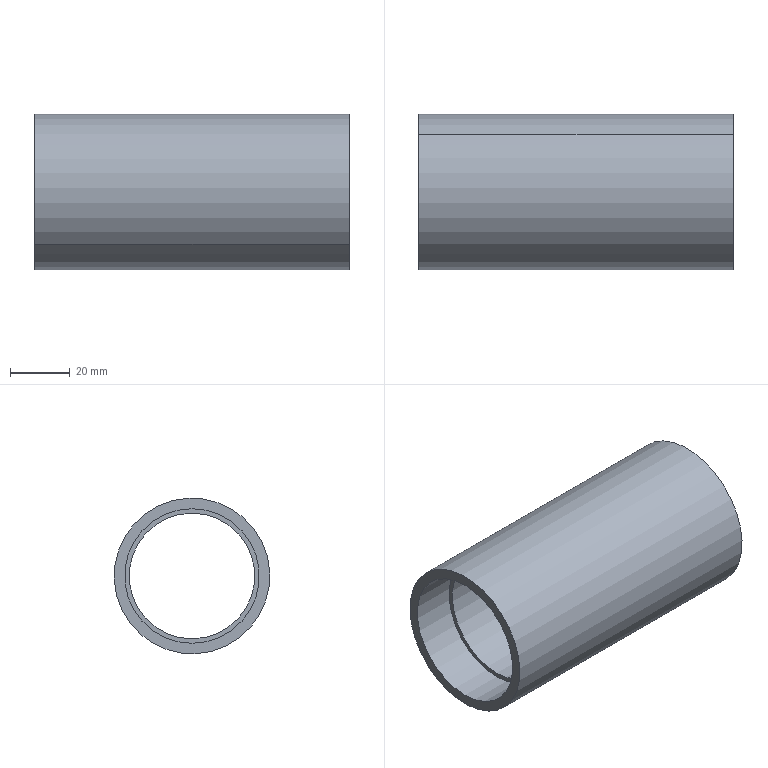Component | SolidWorks | GuideMechanism-1_EncoderRoller-1 | 1 solid | 12 faces | box 105 x 52 x 52 mm | volume 71369 mm3 | cylinder 8 | plane 4 | commonest cylinder face diameters 45 x4 52 x2 42 x2
build123d program:
from build123d import *

# Parameters (mm, degrees)
SKETCH1_W          = 20
SKETCH1_H          = 105
SKETCH2_R          = 21
CUT_EXTRUDE1_DEPTH = 112.252
SKETCH3_R          = 22.5
CUT_EXTRUDE2_DEPTH = 15
CUT_EXTRUDE3_START = -15
SKETCH4_R          = 22.5
CUT_EXTRUDE3_DEPTH = 15


with BuildPart() as part:
    # Sketch1 → Revolve1 (revolve)
    with BuildSketch(Plane.XY):
        with Locations((16, 52.5)):
            Rectangle(SKETCH1_W, SKETCH1_H)
    revolve(axis=Axis((0, -318.491, 0), (0, 1, 0)))

    # Sketch2 → Cut-Extrude1 (cut, through all)
    with BuildSketch(Plane.XZ):
        Circle(SKETCH2_R)
    extrude(amount=-CUT_EXTRUDE1_DEPTH, mode=Mode.SUBTRACT)

    # Sketch3 → Cut-Extrude2 (cut)
    with BuildSketch(Plane.XZ):
        Circle(SKETCH3_R)
    extrude(amount=-CUT_EXTRUDE2_DEPTH, mode=Mode.SUBTRACT)

    # Sketch4 → Cut-Extrude3 (cut)
    with BuildSketch(Plane(origin=(0, 105, 0), x_dir=(1, 0, 0), z_dir=(0, 1, 0)).offset(CUT_EXTRUDE3_START)):
        Circle(SKETCH4_R)
    extrude(amount=CUT_EXTRUDE3_DEPTH, mode=Mode.SUBTRACT)


solid = part.part

# Placed as in the assembly
solid = solid.moved(Location((-386.772, -352.564, 1209.912), (0, 0, 90)))
STEP:
#1=COLOUR_RGB('',0.7922,0.8196,0.9333);
#2=FILL_AREA_STYLE_COLOUR('',#1);
#3=FILL_AREA_STYLE('',(#2));
#4=SURFACE_STYLE_FILL_AREA(#3);
#5=SURFACE_SIDE_STYLE('',(#4));
#6=SURFACE_STYLE_USAGE(.BOTH.,#5);
#7=PRESENTATION_STYLE_ASSIGNMENT((#6));
#8=CARTESIAN_POINT('',(-15.818,-14.538,47.041));
#9=VERTEX_POINT('',#8);
#10=CARTESIAN_POINT('',(-15.818,-13.223,48.227));
#11=VERTEX_POINT('',#10);
#12=CARTESIAN_POINT('',(-15.818,-13.88,47.634));
#13=DIRECTION('',(1.,0.,0.));
#14=DIRECTION('',(0.,0.7428,0.6696));
#15=AXIS2_PLACEMENT_3D('',#12,#13,#14);
#16=CIRCLE('',#15,0.8858);
#17=EDGE_CURVE('',#9,#11,#16,.T.);
#18=ORIENTED_EDGE('',*,*,#17,.F.);
#19=CARTESIAN_POINT('',(-15.227,-14.538,47.041));
#20=VERTEX_POINT('',#19);
#21=CARTESIAN_POINT('',(-15.818,-14.538,47.041));
#22=DIRECTION('',(1.,0.,0.));
#23=VECTOR('',#22,39.37);
#24=LINE('',#21,#23);
#25=EDGE_CURVE('',#9,#20,#24,.T.);
#26=ORIENTED_EDGE('',*,*,#25,.T.);
#27=CARTESIAN_POINT('',(-15.227,-13.223,48.227));
#28=VERTEX_POINT('',#27);
#29=CARTESIAN_POINT('',(-15.227,-13.88,47.634));
#30=DIRECTION('',(1.,0.,0.));
#31=DIRECTION('',(0.,0.7428,0.6696));
#32=AXIS2_PLACEMENT_3D('',#29,#30,#31);
#33=CIRCLE('',#32,0.8858);
#34=EDGE_CURVE('',#20,#28,#33,.T.);
#35=ORIENTED_EDGE('',*,*,#34,.T.);
#36=CARTESIAN_POINT('',(-15.818,-13.223,48.227));
#37=DIRECTION('',(1.,0.,0.));
#38=VECTOR('',#37,39.37);
#39=LINE('',#36,#38);
#40=EDGE_CURVE('',#11,#28,#39,.T.);
#41=ORIENTED_EDGE('',*,*,#40,.F.);
#42=EDGE_LOOP('',(#18,#26,#35,#41));
#43=FACE_OUTER_BOUND('',#42,.T.);
#44=CARTESIAN_POINT('',(-15.818,-13.88,47.634));
#45=DIRECTION('',(1.,0.,0.));
#46=DIRECTION('',(0.,0.7428,0.6696));
#47=AXIS2_PLACEMENT_3D('',#44,#45,#46);
#48=CYLINDRICAL_SURFACE('',#47,0.8858);
#49=ADVANCED_FACE('',(#43),#48,.F.);
#50=CARTESIAN_POINT('',(-18.771,-13.223,48.227));
#51=VERTEX_POINT('',#50);
#52=CARTESIAN_POINT('',(-18.771,-14.538,47.041));
#53=VERTEX_POINT('',#52);
#54=CARTESIAN_POINT('',(-18.771,-13.88,47.634));
#55=DIRECTION('',(-1.,-0.,-0.));
#56=DIRECTION('',(0.,-0.7428,-0.6696));
#57=AXIS2_PLACEMENT_3D('',#54,#55,#56);
#58=CIRCLE('',#57,0.8858);
#59=EDGE_CURVE('',#51,#53,#58,.T.);
#60=ORIENTED_EDGE('',*,*,#59,.F.);
#61=CARTESIAN_POINT('',(-19.361,-13.223,48.227));
#62=VERTEX_POINT('',#61);
#63=CARTESIAN_POINT('',(-18.771,-13.223,48.227));
#64=DIRECTION('',(-1.,-0.,-0.));
#65=VECTOR('',#64,39.37);
#66=LINE('',#63,#65);
#67=EDGE_CURVE('',#51,#62,#66,.T.);
#68=ORIENTED_EDGE('',*,*,#67,.T.);
#69=CARTESIAN_POINT('',(-19.361,-14.538,47.041));
#70=VERTEX_POINT('',#69);
#71=CARTESIAN_POINT('',(-19.361,-13.88,47.634));
#72=DIRECTION('',(-1.,-0.,-0.));
#73=DIRECTION('',(0.,-0.7428,-0.6696));
#74=AXIS2_PLACEMENT_3D('',#71,#72,#73);
#75=CIRCLE('',#74,0.8858);
#76=EDGE_CURVE('',#62,#70,#75,.T.);
#77=ORIENTED_EDGE('',*,*,#76,.T.);
#78=CARTESIAN_POINT('',(-18.771,-14.538,47.041));
#79=DIRECTION('',(-1.,-0.,-0.));
#80=VECTOR('',#79,39.37);
#81=LINE('',#78,#80);
#82=EDGE_CURVE('',#53,#70,#81,.T.);
#83=ORIENTED_EDGE('',*,*,#82,.F.);
#84=EDGE_LOOP('',(#60,#68,#77,#83));
#85=FACE_OUTER_BOUND('',#84,.T.);
#86=CARTESIAN_POINT('',(-18.771,-13.88,47.634));
#87=DIRECTION('',(-1.,-0.,-0.));
#88=DIRECTION('',(0.,-0.7428,-0.6696));
#89=AXIS2_PLACEMENT_3D('',#86,#87,#88);
#90=CYLINDRICAL_SURFACE('',#89,0.8858);
#91=ADVANCED_FACE('',(#85),#90,.F.);
#92=CARTESIAN_POINT('',(-15.227,-14.641,46.949));
#93=VERTEX_POINT('',#92);
#94=CARTESIAN_POINT('',(-15.227,-13.12,48.32));
#95=VERTEX_POINT('',#94);
#96=CARTESIAN_POINT('',(-15.227,-13.88,47.634));
#97=DIRECTION('',(-1.,-0.,-0.));
#98=DIRECTION('',(0.,-0.7428,-0.6696));
#99=AXIS2_PLACEMENT_3D('',#96,#97,#98);
#100=CIRCLE('',#99,1.024);
#101=EDGE_CURVE('',#93,#95,#100,.T.);
#102=ORIENTED_EDGE('',*,*,#101,.T.);
#103=CARTESIAN_POINT('',(-19.361,-13.12,48.32));
#104=VERTEX_POINT('',#103);
#105=CARTESIAN_POINT('',(-31.9,-13.12,48.32));
#106=DIRECTION('',(-1.,-0.,-0.));
#107=VECTOR('',#106,39.37);
#108=LINE('',#105,#107);
#109=EDGE_CURVE('',#95,#104,#108,.T.);
#110=ORIENTED_EDGE('',*,*,#109,.T.);
#111=CARTESIAN_POINT('',(-19.361,-14.641,46.949));
#112=VERTEX_POINT('',#111);
#113=CARTESIAN_POINT('',(-19.361,-13.88,47.634));
#114=DIRECTION('',(-1.,-0.,-0.));
#115=DIRECTION('',(0.,-0.7428,-0.6696));
#116=AXIS2_PLACEMENT_3D('',#113,#114,#115);
#117=CIRCLE('',#116,1.024);
#118=EDGE_CURVE('',#112,#104,#117,.T.);
#119=ORIENTED_EDGE('',*,*,#118,.F.);
#120=CARTESIAN_POINT('',(-31.9,-14.641,46.949));
#121=DIRECTION('',(-1.,-0.,-0.));
#122=VECTOR('',#121,39.37);
#123=LINE('',#120,#122);
#124=EDGE_CURVE('',#93,#112,#123,.T.);
#125=ORIENTED_EDGE('',*,*,#124,.F.);
#126=EDGE_LOOP('',(#102,#110,#119,#125));
#127=FACE_OUTER_BOUND('',#126,.T.);
#128=CARTESIAN_POINT('',(-31.9,-13.88,47.634));
#129=DIRECTION('',(-1.,-0.,-0.));
#130=DIRECTION('',(0.,-0.7428,-0.6696));
#131=AXIS2_PLACEMENT_3D('',#128,#129,#130);
#132=CYLINDRICAL_SURFACE('',#131,1.024);
#133=ADVANCED_FACE('',(#127),#132,.T.);
#134=CARTESIAN_POINT('',(-15.818,-13.266,48.188));
#135=VERTEX_POINT('',#134);
#136=CARTESIAN_POINT('',(-15.818,-14.495,47.081));
#137=VERTEX_POINT('',#136);
#138=CARTESIAN_POINT('',(-15.818,-13.88,47.634));
#139=DIRECTION('',(-1.,-0.,-0.));
#140=DIRECTION('',(0.,0.7428,0.6696));
#141=AXIS2_PLACEMENT_3D('',#138,#139,#140);
#142=CIRCLE('',#141,0.8268);
#143=EDGE_CURVE('',#135,#137,#142,.T.);
#144=ORIENTED_EDGE('',*,*,#143,.F.);
#145=CARTESIAN_POINT('',(-18.771,-13.266,48.188));
#146=VERTEX_POINT('',#145);
#147=CARTESIAN_POINT('',(-15.227,-13.266,48.188));
#148=DIRECTION('',(-1.,-0.,-0.));
#149=VECTOR('',#148,39.37);
#150=LINE('',#147,#149);
#151=EDGE_CURVE('',#135,#146,#150,.T.);
#152=ORIENTED_EDGE('',*,*,#151,.T.);
#153=CARTESIAN_POINT('',(-18.771,-14.495,47.081));
#154=VERTEX_POINT('',#153);
#155=CARTESIAN_POINT('',(-18.771,-13.88,47.634));
#156=DIRECTION('',(1.,0.,0.));
#157=DIRECTION('',(0.,-0.7428,-0.6696));
#158=AXIS2_PLACEMENT_3D('',#155,#156,#157);
#159=CIRCLE('',#158,0.8268);
#160=EDGE_CURVE('',#154,#146,#159,.T.);
#161=ORIENTED_EDGE('',*,*,#160,.F.);
#162=CARTESIAN_POINT('',(-15.227,-14.495,47.081));
#163=DIRECTION('',(-1.,-0.,-0.));
#164=VECTOR('',#163,39.37);
#165=LINE('',#162,#164);
#166=EDGE_CURVE('',#137,#154,#165,.T.);
#167=ORIENTED_EDGE('',*,*,#166,.F.);
#168=EDGE_LOOP('',(#144,#152,#161,#167));
#169=FACE_OUTER_BOUND('',#168,.T.);
#170=CARTESIAN_POINT('',(-15.227,-13.88,47.634));
#171=DIRECTION('',(-1.,-0.,-0.));
#172=DIRECTION('',(0.,-0.7428,-0.6696));
#173=AXIS2_PLACEMENT_3D('',#170,#171,#172);
#174=CYLINDRICAL_SURFACE('',#173,0.8268);
#175=ADVANCED_FACE('',(#169),#174,.F.);
#176=ORIENTED_EDGE('',*,*,#151,.F.);
#177=CARTESIAN_POINT('',(-15.818,-13.88,47.634));
#178=DIRECTION('',(-1.,-0.,-0.));
#179=DIRECTION('',(0.,0.7428,0.6696));
#180=AXIS2_PLACEMENT_3D('',#177,#178,#179);
#181=CIRCLE('',#180,0.8268);
#182=EDGE_CURVE('',#137,#135,#181,.T.);
#183=ORIENTED_EDGE('',*,*,#182,.F.);
#184=ORIENTED_EDGE('',*,*,#166,.T.);
#185=CARTESIAN_POINT('',(-18.771,-13.88,47.634));
#186=DIRECTION('',(1.,0.,0.));
#187=DIRECTION('',(0.,-0.7428,-0.6696));
#188=AXIS2_PLACEMENT_3D('',#185,#186,#187);
#189=CIRCLE('',#188,0.8268);
#190=EDGE_CURVE('',#146,#154,#189,.T.);
#191=ORIENTED_EDGE('',*,*,#190,.F.);
#192=EDGE_LOOP('',(#176,#183,#184,#191));
#193=FACE_OUTER_BOUND('',#192,.T.);
#194=CARTESIAN_POINT('',(-15.227,-13.88,47.634));
#195=DIRECTION('',(-1.,-0.,-0.));
#196=DIRECTION('',(0.,-0.7428,-0.6696));
#197=AXIS2_PLACEMENT_3D('',#194,#195,#196);
#198=CYLINDRICAL_SURFACE('',#197,0.8268);
#199=ADVANCED_FACE('',(#193),#198,.F.);
#200=CARTESIAN_POINT('',(-15.227,-13.88,47.634));
#201=DIRECTION('',(1.,0.,0.));
#202=DIRECTION('',(0.,0.7428,0.6696));
#203=AXIS2_PLACEMENT_3D('',#200,#201,#202);
#204=CIRCLE('',#203,0.8858);
#205=EDGE_CURVE('',#28,#20,#204,.T.);
#206=ORIENTED_EDGE('',*,*,#205,.F.);
#207=ORIENTED_EDGE('',*,*,#34,.F.);
#208=EDGE_LOOP('',(#206,#207));
#209=FACE_BOUND('',#208,.T.);
#210=ORIENTED_EDGE('',*,*,#101,.F.);
#211=CARTESIAN_POINT('',(-15.227,-13.88,47.634));
#212=DIRECTION('',(-1.,-0.,-0.));
#213=DIRECTION('',(0.,-0.7428,-0.6696));
#214=AXIS2_PLACEMENT_3D('',#211,#212,#213);
#215=CIRCLE('',#214,1.024);
#216=EDGE_CURVE('',#95,#93,#215,.T.);
#217=ORIENTED_EDGE('',*,*,#216,.F.);
#218=EDGE_LOOP('',(#210,#217));
#219=FACE_OUTER_BOUND('',#218,.T.);
#220=CARTESIAN_POINT('',(-15.227,-14.641,46.949));
#221=DIRECTION('',(1.,0.,0.));
#222=DIRECTION('',(-0.,0.7428,0.6696));
#223=AXIS2_PLACEMENT_3D('',#220,#221,#222);
#224=PLANE('',#223);
#225=ADVANCED_FACE('',(#209,#219),#224,.T.);
#226=CARTESIAN_POINT('',(-19.361,-13.88,47.634));
#227=DIRECTION('',(-1.,-0.,-0.));
#228=DIRECTION('',(0.,-0.7428,-0.6696));
#229=AXIS2_PLACEMENT_3D('',#226,#227,#228);
#230=CIRCLE('',#229,0.8858);
#231=EDGE_CURVE('',#70,#62,#230,.T.);
#232=ORIENTED_EDGE('',*,*,#231,.F.);
#233=ORIENTED_EDGE('',*,*,#76,.F.);
#234=EDGE_LOOP('',(#232,#233));
#235=FACE_BOUND('',#234,.T.);
#236=ORIENTED_EDGE('',*,*,#118,.T.);
#237=CARTESIAN_POINT('',(-19.361,-13.88,47.634));
#238=DIRECTION('',(-1.,-0.,-0.));
#239=DIRECTION('',(0.,-0.7428,-0.6696));
#240=AXIS2_PLACEMENT_3D('',#237,#238,#239);
#241=CIRCLE('',#240,1.024);
#242=EDGE_CURVE('',#104,#112,#241,.T.);
#243=ORIENTED_EDGE('',*,*,#242,.T.);
#244=EDGE_LOOP('',(#236,#243));
#245=FACE_OUTER_BOUND('',#244,.T.);
#246=CARTESIAN_POINT('',(-19.361,-14.056,47.476));
#247=DIRECTION('',(-1.,-0.,-0.));
#248=DIRECTION('',(0.,-0.7428,-0.6696));
#249=AXIS2_PLACEMENT_3D('',#246,#247,#248);
#250=PLANE('',#249);
#251=ADVANCED_FACE('',(#235,#245),#250,.T.);
#252=ORIENTED_EDGE('',*,*,#109,.F.);
#253=ORIENTED_EDGE('',*,*,#216,.T.);
#254=ORIENTED_EDGE('',*,*,#124,.T.);
#255=ORIENTED_EDGE('',*,*,#242,.F.);
#256=EDGE_LOOP('',(#252,#253,#254,#255));
#257=FACE_OUTER_BOUND('',#256,.T.);
#258=CARTESIAN_POINT('',(-31.9,-13.88,47.634));
#259=DIRECTION('',(-1.,-0.,-0.));
#260=DIRECTION('',(0.,-0.7428,-0.6696));
#261=AXIS2_PLACEMENT_3D('',#258,#259,#260);
#262=CYLINDRICAL_SURFACE('',#261,1.024);
#263=ADVANCED_FACE('',(#257),#262,.T.);
#264=CARTESIAN_POINT('',(-18.771,-13.88,47.634));
#265=DIRECTION('',(-1.,-0.,-0.));
#266=DIRECTION('',(0.,-0.7428,-0.6696));
#267=AXIS2_PLACEMENT_3D('',#264,#265,#266);
#268=CIRCLE('',#267,0.8858);
#269=EDGE_CURVE('',#53,#51,#268,.T.);
#270=ORIENTED_EDGE('',*,*,#269,.T.);
#271=ORIENTED_EDGE('',*,*,#59,.T.);
#272=EDGE_LOOP('',(#270,#271));
#273=FACE_OUTER_BOUND('',#272,.T.);
#274=ORIENTED_EDGE('',*,*,#160,.T.);
#275=ORIENTED_EDGE('',*,*,#190,.T.);
#276=EDGE_LOOP('',(#274,#275));
#277=FACE_BOUND('',#276,.T.);
#278=CARTESIAN_POINT('',(-18.771,-13.88,47.634));
#279=DIRECTION('',(-1.,-0.,-0.));
#280=DIRECTION('',(0.,-0.7428,-0.6696));
#281=AXIS2_PLACEMENT_3D('',#278,#279,#280);
#282=PLANE('',#281);
#283=ADVANCED_FACE('',(#273,#277),#282,.T.);
#284=ORIENTED_EDGE('',*,*,#67,.F.);
#285=ORIENTED_EDGE('',*,*,#269,.F.);
#286=ORIENTED_EDGE('',*,*,#82,.T.);
#287=ORIENTED_EDGE('',*,*,#231,.T.);
#288=EDGE_LOOP('',(#284,#285,#286,#287));
#289=FACE_OUTER_BOUND('',#288,.T.);
#290=CARTESIAN_POINT('',(-18.771,-13.88,47.634));
#291=DIRECTION('',(-1.,-0.,-0.));
#292=DIRECTION('',(0.,-0.7428,-0.6696));
#293=AXIS2_PLACEMENT_3D('',#290,#291,#292);
#294=CYLINDRICAL_SURFACE('',#293,0.8858);
#295=ADVANCED_FACE('',(#289),#294,.F.);
#296=CARTESIAN_POINT('',(-15.818,-13.88,47.634));
#297=DIRECTION('',(1.,0.,0.));
#298=DIRECTION('',(0.,0.7428,0.6696));
#299=AXIS2_PLACEMENT_3D('',#296,#297,#298);
#300=CIRCLE('',#299,0.8858);
#301=EDGE_CURVE('',#11,#9,#300,.T.);
#302=ORIENTED_EDGE('',*,*,#301,.T.);
#303=ORIENTED_EDGE('',*,*,#17,.T.);
#304=EDGE_LOOP('',(#302,#303));
#305=FACE_OUTER_BOUND('',#304,.T.);
#306=ORIENTED_EDGE('',*,*,#182,.T.);
#307=ORIENTED_EDGE('',*,*,#143,.T.);
#308=EDGE_LOOP('',(#306,#307));
#309=FACE_BOUND('',#308,.T.);
#310=CARTESIAN_POINT('',(-15.818,-13.88,47.634));
#311=DIRECTION('',(1.,0.,0.));
#312=DIRECTION('',(-0.,0.7428,0.6696));
#313=AXIS2_PLACEMENT_3D('',#310,#311,#312);
#314=PLANE('',#313);
#315=ADVANCED_FACE('',(#305,#309),#314,.T.);
#316=ORIENTED_EDGE('',*,*,#25,.F.);
#317=ORIENTED_EDGE('',*,*,#301,.F.);
#318=ORIENTED_EDGE('',*,*,#40,.T.);
#319=ORIENTED_EDGE('',*,*,#205,.T.);
#320=EDGE_LOOP('',(#316,#317,#318,#319));
#321=FACE_OUTER_BOUND('',#320,.T.);
#322=CARTESIAN_POINT('',(-15.818,-13.88,47.634));
#323=DIRECTION('',(1.,0.,0.));
#324=DIRECTION('',(0.,0.7428,0.6696));
#325=AXIS2_PLACEMENT_3D('',#322,#323,#324);
#326=CYLINDRICAL_SURFACE('',#325,0.8858);
#327=ADVANCED_FACE('',(#321),#326,.F.);
#328=CLOSED_SHELL('',(#49,#91,#133,#175,#199,#225,#251,#263,#283,#295,#315,#327));
#329=MANIFOLD_SOLID_BREP('',#328);
#330=STYLED_ITEM('',(#7),#329);
#331=(LENGTH_UNIT()NAMED_UNIT(*)SI_UNIT($,.METRE.));
#332=LENGTH_MEASURE_WITH_UNIT(LENGTH_MEASURE(0.0254),#331);
#333=DIMENSIONAL_EXPONENTS(1.,0.,0.,0.,0.,0.,0.);
#334=(CONVERSION_BASED_UNIT('',#332)LENGTH_UNIT()NAMED_UNIT(#333));
#335=UNCERTAINTY_MEASURE_WITH_UNIT(LENGTH_MEASURE(0.00001),#334,'','');
#336=(NAMED_UNIT(*)PLANE_ANGLE_UNIT()SI_UNIT($,.RADIAN.));
#337=(NAMED_UNIT(*)SI_UNIT($,.STERADIAN.)SOLID_ANGLE_UNIT());
#338=(GEOMETRIC_REPRESENTATION_CONTEXT(3)GLOBAL_UNCERTAINTY_ASSIGNED_CONTEXT((#335))GLOBAL_UNIT_ASSIGNED_CONTEXT((#334,#336,#337))REPRESENTATION_CONTEXT('',''));
#339=MECHANICAL_DESIGN_GEOMETRIC_PRESENTATION_REPRESENTATION('',(#330),#338);
#340=CARTESIAN_POINT('',(0.,0.,0.));
#341=DIRECTION('',(0.,0.,1.));
#342=DIRECTION('',(1.,0.,0.));
#343=AXIS2_PLACEMENT_3D('',#340,#341,#342);
#344=(LENGTH_UNIT()NAMED_UNIT(*)SI_UNIT($,.METRE.));
#345=LENGTH_MEASURE_WITH_UNIT(LENGTH_MEASURE(0.0254),#344);
#346=DIMENSIONAL_EXPONENTS(1.,0.,0.,0.,0.,0.,0.);
#347=(CONVERSION_BASED_UNIT('',#345)LENGTH_UNIT()NAMED_UNIT(#346));
#348=UNCERTAINTY_MEASURE_WITH_UNIT(LENGTH_MEASURE(0.00001),#347,'','');
#349=(NAMED_UNIT(*)PLANE_ANGLE_UNIT()SI_UNIT($,.RADIAN.));
#350=(NAMED_UNIT(*)SI_UNIT($,.STERADIAN.)SOLID_ANGLE_UNIT());
#351=(GEOMETRIC_REPRESENTATION_CONTEXT(3)GLOBAL_UNCERTAINTY_ASSIGNED_CONTEXT((#348))GLOBAL_UNIT_ASSIGNED_CONTEXT((#347,#349,#350))REPRESENTATION_CONTEXT('',''));
#352=ADVANCED_BREP_SHAPE_REPRESENTATION('',(#329,#343),#351);
#353=PRESENTATION_LAYER_ASSIGNMENT('','',(#330));